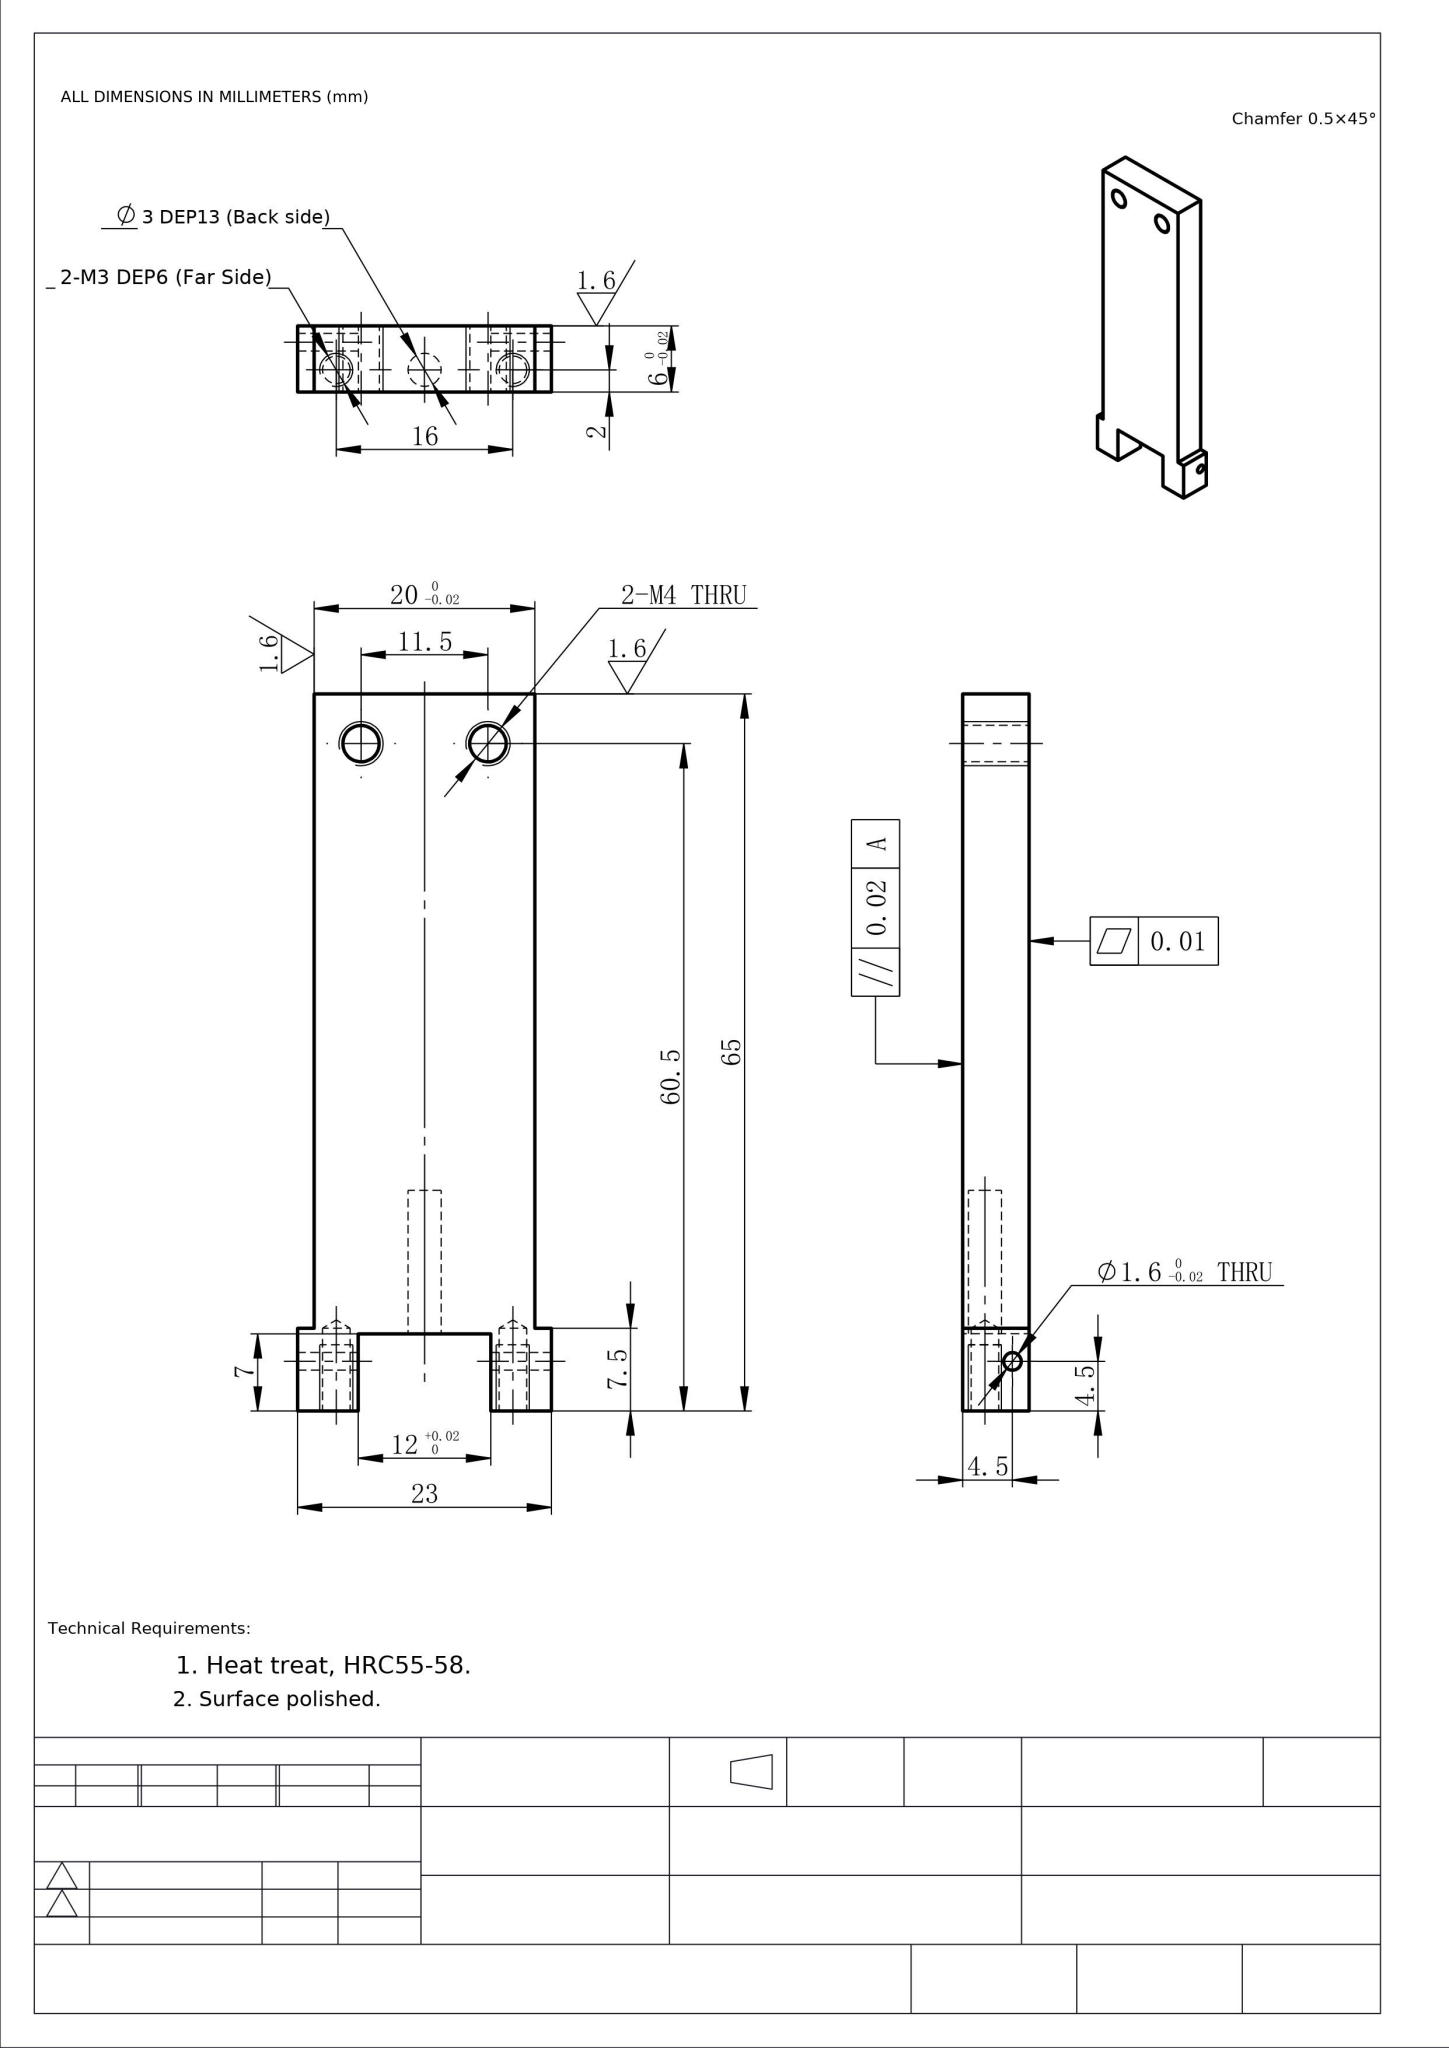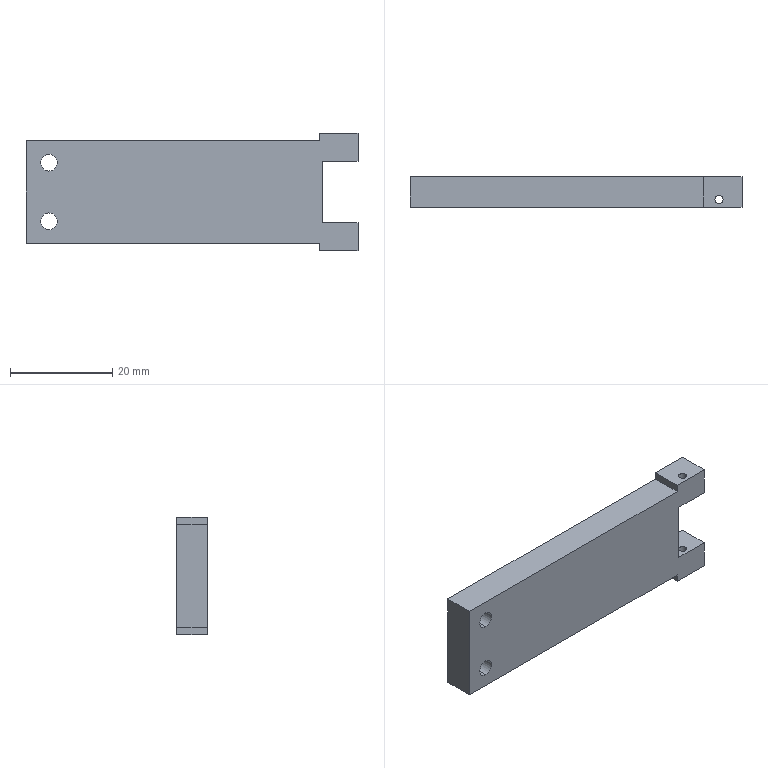Part | NX | mm | 1 solid | 33 faces | box 65 x 6 x 23 mm | volume 7138 mm3 | plane 15 | cylinder 14 | cone 4 | commonest cylinder face diameters 1.6 x4 2.5 x4 3.3 x4 3 x2